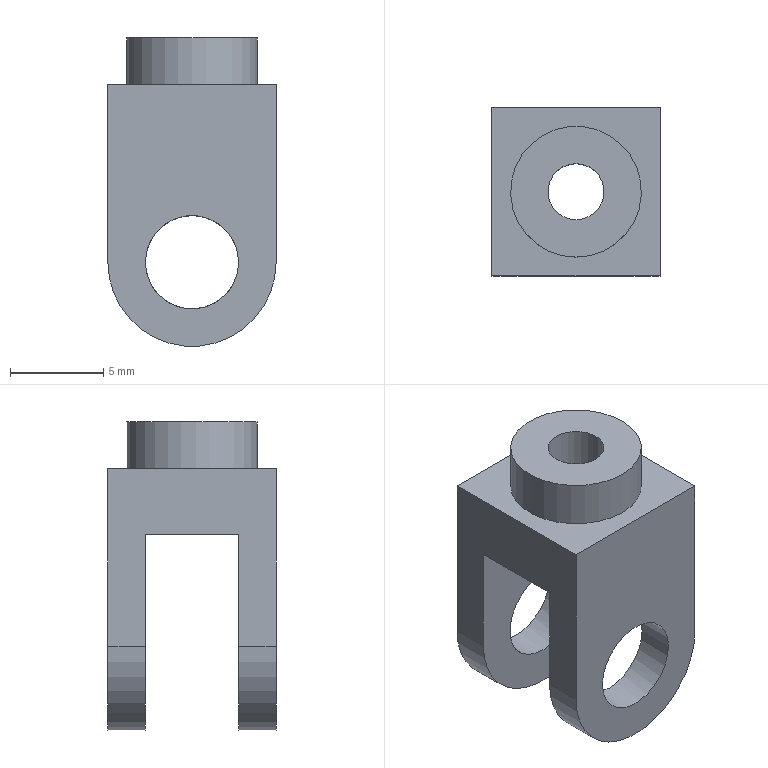Component | NX | CONN_BLOCK | 1 solid | 15 faces | box 9 x 9 x 16.5 mm | volume 602 mm3 | plane 9 | cylinder 6 | commonest cylinder face diameters 9 x2 5 x2 7 x1 3 x1
STEP:
#1=CARTESIAN_POINT('',(0.,0.,0.));
#2=DIRECTION('',(0.,0.,1.));
#3=DIRECTION('',(1.,0.,0.));
#4=AXIS2_PLACEMENT_3D('',#1,#2,#3);
#5=CARTESIAN_POINT('',(-4.5,18.5,86.631));
#6=VERTEX_POINT('',#5);
#7=CARTESIAN_POINT('',(-4.5,20.5,86.631));
#8=VERTEX_POINT('',#7);
#9=CARTESIAN_POINT('',(-4.5,18.5,86.631));
#10=DIRECTION('',(0.,1.,0.));
#11=VECTOR('',#10,1.);
#12=LINE('',#9,#11);
#13=CARTESIAN_POINT('',(-0.,18.5,86.631));
#14=DIRECTION('',(0.,1.,0.));
#15=DIRECTION('',(0.,0.,1.));
#16=AXIS2_PLACEMENT_3D('',#13,#14,#15);
#17=CYLINDRICAL_SURFACE('',#16,4.5);
#18=CARTESIAN_POINT('',(4.712,0.));
#19=DIRECTION('',(0.,1.));
#20=VECTOR('',#19,1.);
#21=LINE('',#18,#20);
#22=(GEOMETRIC_REPRESENTATION_CONTEXT(2)PARAMETRIC_REPRESENTATION_CONTEXT()REPRESENTATION_CONTEXT('',''));
#23=DEFINITIONAL_REPRESENTATION('',(#21),#22);
#24=PCURVE('',#17,#23);
#25=CARTESIAN_POINT('',(-4.5,18.5,96.131));
#26=DIRECTION('',(1.,0.,0.));
#27=DIRECTION('',(-0.,0.,1.));
#28=AXIS2_PLACEMENT_3D('',#25,#26,#27);
#29=PLANE('',#28);
#30=CARTESIAN_POINT('',(-9.5,0.));
#31=DIRECTION('',(0.,-1.));
#32=VECTOR('',#31,1.);
#33=LINE('',#30,#32);
#34=(GEOMETRIC_REPRESENTATION_CONTEXT(2)PARAMETRIC_REPRESENTATION_CONTEXT()REPRESENTATION_CONTEXT('',''));
#35=DEFINITIONAL_REPRESENTATION('',(#33),#34);
#36=PCURVE('',#29,#35);
#37=SURFACE_CURVE('',#12,(#24,#36),.PCURVE_S1.);
#38=EDGE_CURVE('',#6,#8,#37,.T.);
#39=ORIENTED_EDGE('',*,*,#38,.T.);
#40=CARTESIAN_POINT('',(4.5,20.5,86.631));
#41=VERTEX_POINT('',#40);
#42=CARTESIAN_POINT('',(-0.,20.5,86.631));
#43=DIRECTION('',(0.,-1.,-0.));
#44=DIRECTION('',(0.,0.,-1.));
#45=AXIS2_PLACEMENT_3D('',#42,#43,#44);
#46=CIRCLE('',#45,4.5);
#47=CARTESIAN_POINT('',(9.425,2.));
#48=DIRECTION('',(-1.,0.));
#49=VECTOR('',#48,1.);
#50=LINE('',#47,#49);
#51=(GEOMETRIC_REPRESENTATION_CONTEXT(2)PARAMETRIC_REPRESENTATION_CONTEXT()REPRESENTATION_CONTEXT('',''));
#52=DEFINITIONAL_REPRESENTATION('',(#50),#51);
#53=PCURVE('',#17,#52);
#54=CARTESIAN_POINT('',(-5.,20.5,92.631));
#55=DIRECTION('',(0.,-1.,-0.));
#56=DIRECTION('',(0.,0.,-1.));
#57=AXIS2_PLACEMENT_3D('',#54,#55,#56);
#58=PLANE('',#57);
#59=CARTESIAN_POINT('',(6.,5.));
#60=DIRECTION('',(1.,0.));
#61=AXIS2_PLACEMENT_2D('',#59,#60);
#62=CIRCLE('',#61,4.5);
#63=(GEOMETRIC_REPRESENTATION_CONTEXT(2)PARAMETRIC_REPRESENTATION_CONTEXT()REPRESENTATION_CONTEXT('',''));
#64=DEFINITIONAL_REPRESENTATION('',(#62),#63);
#65=PCURVE('',#58,#64);
#66=SURFACE_CURVE('',#46,(#53,#65),.PCURVE_S1.);
#67=EDGE_CURVE('',#8,#41,#66,.T.);
#68=ORIENTED_EDGE('',*,*,#67,.T.);
#69=CARTESIAN_POINT('',(4.5,18.5,86.631));
#70=VERTEX_POINT('',#69);
#71=CARTESIAN_POINT('',(4.5,18.5,86.631));
#72=DIRECTION('',(0.,1.,0.));
#73=VECTOR('',#72,1.);
#74=LINE('',#71,#73);
#75=CARTESIAN_POINT('',(1.571,0.));
#76=DIRECTION('',(0.,1.));
#77=VECTOR('',#76,1.);
#78=LINE('',#75,#77);
#79=(GEOMETRIC_REPRESENTATION_CONTEXT(2)PARAMETRIC_REPRESENTATION_CONTEXT()REPRESENTATION_CONTEXT('',''));
#80=DEFINITIONAL_REPRESENTATION('',(#78),#79);
#81=PCURVE('',#17,#80);
#82=CARTESIAN_POINT('',(4.5,18.5,86.631));
#83=DIRECTION('',(-1.,0.,0.));
#84=DIRECTION('',(-0.,0.,-1.));
#85=AXIS2_PLACEMENT_3D('',#82,#83,#84);
#86=PLANE('',#85);
#87=CARTESIAN_POINT('',(0.,0.));
#88=DIRECTION('',(0.,-1.));
#89=VECTOR('',#88,1.);
#90=LINE('',#87,#89);
#91=(GEOMETRIC_REPRESENTATION_CONTEXT(2)PARAMETRIC_REPRESENTATION_CONTEXT()REPRESENTATION_CONTEXT('',''));
#92=DEFINITIONAL_REPRESENTATION('',(#90),#91);
#93=PCURVE('',#86,#92);
#94=SURFACE_CURVE('',#74,(#81,#93),.PCURVE_S1.);
#95=EDGE_CURVE('',#70,#41,#94,.T.);
#96=ORIENTED_EDGE('',*,*,#95,.F.);
#97=CARTESIAN_POINT('',(-0.,18.5,86.631));
#98=DIRECTION('',(0.,-1.,0.));
#99=DIRECTION('',(1.,0.,0.));
#100=AXIS2_PLACEMENT_3D('',#97,#98,#99);
#101=CIRCLE('',#100,4.5);
#102=CARTESIAN_POINT('',(7.854,0.));
#103=DIRECTION('',(-1.,0.));
#104=VECTOR('',#103,1.);
#105=LINE('',#102,#104);
#106=(GEOMETRIC_REPRESENTATION_CONTEXT(2)PARAMETRIC_REPRESENTATION_CONTEXT()REPRESENTATION_CONTEXT('',''));
#107=DEFINITIONAL_REPRESENTATION('',(#105),#106);
#108=PCURVE('',#17,#107);
#109=CARTESIAN_POINT('',(-0.,18.5,86.631));
#110=DIRECTION('',(0.,-1.,0.));
#111=DIRECTION('',(0.,0.,-1.));
#112=AXIS2_PLACEMENT_3D('',#109,#110,#111);
#113=PLANE('',#112);
#114=CARTESIAN_POINT('',(0.,0.));
#115=DIRECTION('',(0.,1.));
#116=AXIS2_PLACEMENT_2D('',#114,#115);
#117=CIRCLE('',#116,4.5);
#118=(GEOMETRIC_REPRESENTATION_CONTEXT(2)PARAMETRIC_REPRESENTATION_CONTEXT()REPRESENTATION_CONTEXT('',''));
#119=DEFINITIONAL_REPRESENTATION('',(#117),#118);
#120=PCURVE('',#113,#119);
#121=SURFACE_CURVE('',#101,(#108,#120),.PCURVE_S1.);
#122=EDGE_CURVE('',#6,#70,#121,.T.);
#123=ORIENTED_EDGE('',*,*,#122,.F.);
#124=EDGE_LOOP('',(#39,#68,#96,#123));
#125=FACE_BOUND('',#124,.T.);
#126=ADVANCED_FACE('',(#125),#17,.T.);
#127=CARTESIAN_POINT('',(-0.,25.5,89.131));
#128=VERTEX_POINT('',#127);
#129=CARTESIAN_POINT('',(-0.,25.5,86.631));
#130=DIRECTION('',(0.,1.,-0.));
#131=DIRECTION('',(0.,0.,1.));
#132=AXIS2_PLACEMENT_3D('',#129,#130,#131);
#133=CIRCLE('',#132,2.5);
#134=CARTESIAN_POINT('',(-0.,18.5,86.631));
#135=DIRECTION('',(0.,1.,0.));
#136=DIRECTION('',(0.,0.,1.));
#137=AXIS2_PLACEMENT_3D('',#134,#135,#136);
#138=CYLINDRICAL_SURFACE('',#137,2.5);
#139=CARTESIAN_POINT('',(0.,7.));
#140=DIRECTION('',(1.,0.));
#141=VECTOR('',#140,1.);
#142=LINE('',#139,#141);
#143=(GEOMETRIC_REPRESENTATION_CONTEXT(2)PARAMETRIC_REPRESENTATION_CONTEXT()REPRESENTATION_CONTEXT('',''));
#144=DEFINITIONAL_REPRESENTATION('',(#142),#143);
#145=PCURVE('',#138,#144);
#146=CARTESIAN_POINT('',(-5.,25.5,82.131));
#147=DIRECTION('',(0.,1.,-0.));
#148=DIRECTION('',(0.,0.,1.));
#149=AXIS2_PLACEMENT_3D('',#146,#147,#148);
#150=PLANE('',#149);
#151=CARTESIAN_POINT('',(4.5,5.));
#152=DIRECTION('',(1.,0.));
#153=AXIS2_PLACEMENT_2D('',#151,#152);
#154=CIRCLE('',#153,2.5);
#155=(GEOMETRIC_REPRESENTATION_CONTEXT(2)PARAMETRIC_REPRESENTATION_CONTEXT()REPRESENTATION_CONTEXT('',''));
#156=DEFINITIONAL_REPRESENTATION('',(#154),#155);
#157=PCURVE('',#150,#156);
#158=SURFACE_CURVE('',#133,(#145,#157),.PCURVE_S1.);
#159=EDGE_CURVE('',#128,#128,#158,.T.);
#160=ORIENTED_EDGE('',*,*,#159,.T.);
#161=CARTESIAN_POINT('',(-0.,27.5,89.131));
#162=VERTEX_POINT('',#161);
#163=CARTESIAN_POINT('',(-0.,25.5,89.131));
#164=CARTESIAN_POINT('',(-0.,27.5,89.131));
#165=B_SPLINE_CURVE_WITH_KNOTS('',1,(#163,#164),.UNSPECIFIED.,.F.,.F.,(2,2),(7.,9.),.PIECEWISE_BEZIER_KNOTS.);
#166=CARTESIAN_POINT('',(6.283,0.));
#167=DIRECTION('',(0.,1.));
#168=VECTOR('',#167,1.);
#169=LINE('',#166,#168);
#170=(GEOMETRIC_REPRESENTATION_CONTEXT(2)PARAMETRIC_REPRESENTATION_CONTEXT()REPRESENTATION_CONTEXT('',''));
#171=DEFINITIONAL_REPRESENTATION('',(#169),#170);
#172=PCURVE('',#138,#171);
#173=CARTESIAN_POINT('',(0.,0.));
#174=DIRECTION('',(0.,1.));
#175=VECTOR('',#174,1.);
#176=LINE('',#173,#175);
#177=(GEOMETRIC_REPRESENTATION_CONTEXT(2)PARAMETRIC_REPRESENTATION_CONTEXT()REPRESENTATION_CONTEXT('',''));
#178=DEFINITIONAL_REPRESENTATION('',(#176),#177);
#179=PCURVE('',#138,#178);
#180=SEAM_CURVE('',#165,(#172,#179),.PCURVE_S1.);
#181=EDGE_CURVE('',#128,#162,#180,.T.);
#182=ORIENTED_EDGE('',*,*,#181,.T.);
#183=CARTESIAN_POINT('',(2.5,27.5,86.631));
#184=VERTEX_POINT('',#183);
#185=CARTESIAN_POINT('',(-0.,27.5,86.631));
#186=DIRECTION('',(0.,-1.,0.));
#187=DIRECTION('',(1.,0.,0.));
#188=AXIS2_PLACEMENT_3D('',#185,#186,#187);
#189=CIRCLE('',#188,2.5);
#190=CARTESIAN_POINT('',(7.854,9.));
#191=DIRECTION('',(-1.,0.));
#192=VECTOR('',#191,1.);
#193=LINE('',#190,#192);
#194=(GEOMETRIC_REPRESENTATION_CONTEXT(2)PARAMETRIC_REPRESENTATION_CONTEXT()REPRESENTATION_CONTEXT('',''));
#195=DEFINITIONAL_REPRESENTATION('',(#193),#194);
#196=PCURVE('',#138,#195);
#197=CARTESIAN_POINT('',(-0.,27.5,86.631));
#198=DIRECTION('',(0.,-1.,0.));
#199=DIRECTION('',(0.,0.,-1.));
#200=AXIS2_PLACEMENT_3D('',#197,#198,#199);
#201=PLANE('',#200);
#202=CARTESIAN_POINT('',(0.,0.));
#203=DIRECTION('',(0.,1.));
#204=AXIS2_PLACEMENT_2D('',#202,#203);
#205=CIRCLE('',#204,2.5);
#206=(GEOMETRIC_REPRESENTATION_CONTEXT(2)PARAMETRIC_REPRESENTATION_CONTEXT()REPRESENTATION_CONTEXT('',''));
#207=DEFINITIONAL_REPRESENTATION('',(#205),#206);
#208=PCURVE('',#201,#207);
#209=SURFACE_CURVE('',#189,(#196,#208),.PCURVE_S1.);
#210=EDGE_CURVE('',#162,#184,#209,.T.);
#211=ORIENTED_EDGE('',*,*,#210,.T.);
#212=CARTESIAN_POINT('',(-0.,27.5,86.631));
#213=DIRECTION('',(0.,-1.,0.));
#214=DIRECTION('',(1.,0.,0.));
#215=AXIS2_PLACEMENT_3D('',#212,#213,#214);
#216=CIRCLE('',#215,2.5);
#217=CARTESIAN_POINT('',(1.571,9.));
#218=DIRECTION('',(-1.,0.));
#219=VECTOR('',#218,1.);
#220=LINE('',#217,#219);
#221=(GEOMETRIC_REPRESENTATION_CONTEXT(2)PARAMETRIC_REPRESENTATION_CONTEXT()REPRESENTATION_CONTEXT('',''));
#222=DEFINITIONAL_REPRESENTATION('',(#220),#221);
#223=PCURVE('',#138,#222);
#224=CARTESIAN_POINT('',(0.,0.));
#225=DIRECTION('',(0.,1.));
#226=AXIS2_PLACEMENT_2D('',#224,#225);
#227=CIRCLE('',#226,2.5);
#228=(GEOMETRIC_REPRESENTATION_CONTEXT(2)PARAMETRIC_REPRESENTATION_CONTEXT()REPRESENTATION_CONTEXT('',''));
#229=DEFINITIONAL_REPRESENTATION('',(#227),#228);
#230=PCURVE('',#201,#229);
#231=SURFACE_CURVE('',#216,(#223,#230),.PCURVE_S1.);
#232=EDGE_CURVE('',#184,#162,#231,.T.);
#233=ORIENTED_EDGE('',*,*,#232,.T.);
#234=ORIENTED_EDGE('',*,*,#181,.F.);
#235=EDGE_LOOP('',(#160,#182,#211,#233,#234));
#236=FACE_BOUND('',#235,.F.);
#237=ADVANCED_FACE('',(#236),#138,.F.);
#238=CARTESIAN_POINT('',(-0.,21.5,98.631));
#239=VERTEX_POINT('',#238);
#240=CARTESIAN_POINT('',(-0.,23.,98.631));
#241=DIRECTION('',(0.,0.,-1.));
#242=DIRECTION('',(0.,-1.,0.));
#243=AXIS2_PLACEMENT_3D('',#240,#241,#242);
#244=CIRCLE('',#243,1.5);
#245=CARTESIAN_POINT('',(-0.,23.,98.631));
#246=DIRECTION('',(0.,0.,1.));
#247=DIRECTION('',(0.,-1.,0.));
#248=AXIS2_PLACEMENT_3D('',#245,#246,#247);
#249=PLANE('',#248);
#250=CARTESIAN_POINT('',(1.5,0.));
#251=CARTESIAN_POINT('',(1.5,-2.598));
#252=CARTESIAN_POINT('',(-0.75,-1.299));
#253=CARTESIAN_POINT('',(-3.,-0.));
#254=CARTESIAN_POINT('',(-0.75,1.299));
#255=CARTESIAN_POINT('',(1.5,2.598));
#256=CARTESIAN_POINT('',(1.5,0.));
#257=(BOUNDED_CURVE()B_SPLINE_CURVE(2,(#250,#251,#252,#253,#254,#255,#256),.UNSPECIFIED.,.T.,.F.)B_SPLINE_CURVE_WITH_KNOTS((1,2,2,2,2,1),(-2.094,0.,2.094,4.189,6.283,8.378),.UNSPECIFIED.)CURVE()GEOMETRIC_REPRESENTATION_ITEM()RATIONAL_B_SPLINE_CURVE((1.,0.5,1.,0.5,1.,0.5,1.))REPRESENTATION_ITEM(''));
#258=(GEOMETRIC_REPRESENTATION_CONTEXT(2)PARAMETRIC_REPRESENTATION_CONTEXT()REPRESENTATION_CONTEXT('',''));
#259=DEFINITIONAL_REPRESENTATION('',(#257),#258);
#260=PCURVE('',#249,#259);
#261=CARTESIAN_POINT('',(-0.,23.,88.131));
#262=DIRECTION('',(0.,0.,1.));
#263=DIRECTION('',(0.,-1.,0.));
#264=AXIS2_PLACEMENT_3D('',#261,#262,#263);
#265=CYLINDRICAL_SURFACE('',#264,1.5);
#266=CARTESIAN_POINT('',(6.283,10.5));
#267=DIRECTION('',(-1.,0.));
#268=VECTOR('',#267,1.);
#269=LINE('',#266,#268);
#270=(GEOMETRIC_REPRESENTATION_CONTEXT(2)PARAMETRIC_REPRESENTATION_CONTEXT()REPRESENTATION_CONTEXT('',''));
#271=DEFINITIONAL_REPRESENTATION('',(#269),#270);
#272=PCURVE('',#265,#271);
#273=SURFACE_CURVE('',#244,(#260,#272),.PCURVE_S1.);
#274=EDGE_CURVE('',#239,#239,#273,.T.);
#275=ORIENTED_EDGE('',*,*,#274,.T.);
#276=EDGE_LOOP('',(#275));
#277=FACE_BOUND('',#276,.T.);
#278=CARTESIAN_POINT('',(-0.,19.5,98.631));
#279=VERTEX_POINT('',#278);
#280=CARTESIAN_POINT('',(-0.,23.,98.631));
#281=DIRECTION('',(0.,0.,-1.));
#282=DIRECTION('',(0.,-1.,0.));
#283=AXIS2_PLACEMENT_3D('',#280,#281,#282);
#284=CIRCLE('',#283,3.5);
#285=CARTESIAN_POINT('',(3.5,0.));
#286=CARTESIAN_POINT('',(3.5,-6.062));
#287=CARTESIAN_POINT('',(-1.75,-3.031));
#288=CARTESIAN_POINT('',(-7.,-0.));
#289=CARTESIAN_POINT('',(-1.75,3.031));
#290=CARTESIAN_POINT('',(3.5,6.062));
#291=CARTESIAN_POINT('',(3.5,0.));
#292=(BOUNDED_CURVE()B_SPLINE_CURVE(2,(#285,#286,#287,#288,#289,#290,#291),.UNSPECIFIED.,.T.,.F.)B_SPLINE_CURVE_WITH_KNOTS((1,2,2,2,2,1),(-2.094,0.,2.094,4.189,6.283,8.378),.UNSPECIFIED.)CURVE()GEOMETRIC_REPRESENTATION_ITEM()RATIONAL_B_SPLINE_CURVE((1.,0.5,1.,0.5,1.,0.5,1.))REPRESENTATION_ITEM(''));
#293=(GEOMETRIC_REPRESENTATION_CONTEXT(2)PARAMETRIC_REPRESENTATION_CONTEXT()REPRESENTATION_CONTEXT('',''));
#294=DEFINITIONAL_REPRESENTATION('',(#292),#293);
#295=PCURVE('',#249,#294);
#296=CARTESIAN_POINT('',(-0.,23.,96.131));
#297=DIRECTION('',(0.,0.,1.));
#298=DIRECTION('',(0.,-1.,0.));
#299=AXIS2_PLACEMENT_3D('',#296,#297,#298);
#300=CYLINDRICAL_SURFACE('',#299,3.5);
#301=CARTESIAN_POINT('',(6.283,2.5));
#302=DIRECTION('',(-1.,0.));
#303=VECTOR('',#302,1.);
#304=LINE('',#301,#303);
#305=(GEOMETRIC_REPRESENTATION_CONTEXT(2)PARAMETRIC_REPRESENTATION_CONTEXT()REPRESENTATION_CONTEXT('',''));
#306=DEFINITIONAL_REPRESENTATION('',(#304),#305);
#307=PCURVE('',#300,#306);
#308=SURFACE_CURVE('',#284,(#295,#307),.PCURVE_S1.);
#309=EDGE_CURVE('',#279,#279,#308,.T.);
#310=ORIENTED_EDGE('',*,*,#309,.F.);
#311=EDGE_LOOP('',(#310));
#312=FACE_BOUND('',#311,.T.);
#313=ADVANCED_FACE('',(#277,#312),#249,.T.);
#314=ORIENTED_EDGE('',*,*,#309,.T.);
#315=CARTESIAN_POINT('',(-0.,19.5,96.131));
#316=VERTEX_POINT('',#315);
#317=CARTESIAN_POINT('',(-0.,19.5,96.131));
#318=CARTESIAN_POINT('',(-0.,19.5,98.631));
#319=B_SPLINE_CURVE_WITH_KNOTS('',1,(#317,#318),.UNSPECIFIED.,.F.,.F.,(2,2),(0.,2.5),.PIECEWISE_BEZIER_KNOTS.);
#320=CARTESIAN_POINT('',(0.,0.));
#321=DIRECTION('',(0.,1.));
#322=VECTOR('',#321,1.);
#323=LINE('',#320,#322);
#324=(GEOMETRIC_REPRESENTATION_CONTEXT(2)PARAMETRIC_REPRESENTATION_CONTEXT()REPRESENTATION_CONTEXT('',''));
#325=DEFINITIONAL_REPRESENTATION('',(#323),#324);
#326=PCURVE('',#300,#325);
#327=CARTESIAN_POINT('',(6.283,0.));
#328=DIRECTION('',(0.,1.));
#329=VECTOR('',#328,1.);
#330=LINE('',#327,#329);
#331=(GEOMETRIC_REPRESENTATION_CONTEXT(2)PARAMETRIC_REPRESENTATION_CONTEXT()REPRESENTATION_CONTEXT('',''));
#332=DEFINITIONAL_REPRESENTATION('',(#330),#331);
#333=PCURVE('',#300,#332);
#334=SEAM_CURVE('',#319,(#326,#333),.PCURVE_S1.);
#335=EDGE_CURVE('',#316,#279,#334,.T.);
#336=ORIENTED_EDGE('',*,*,#335,.F.);
#337=CARTESIAN_POINT('',(-0.,23.,96.131));
#338=DIRECTION('',(0.,0.,1.));
#339=DIRECTION('',(0.,-1.,0.));
#340=AXIS2_PLACEMENT_3D('',#337,#338,#339);
#341=CIRCLE('',#340,3.5);
#342=CARTESIAN_POINT('',(0.,0.));
#343=DIRECTION('',(1.,0.));
#344=VECTOR('',#343,1.);
#345=LINE('',#342,#344);
#346=(GEOMETRIC_REPRESENTATION_CONTEXT(2)PARAMETRIC_REPRESENTATION_CONTEXT()REPRESENTATION_CONTEXT('',''));
#347=DEFINITIONAL_REPRESENTATION('',(#345),#346);
#348=PCURVE('',#300,#347);
#349=CARTESIAN_POINT('',(-0.,18.5,96.131));
#350=DIRECTION('',(0.,0.,-1.));
#351=DIRECTION('',(0.,1.,0.));
#352=AXIS2_PLACEMENT_3D('',#349,#350,#351);
#353=PLANE('',#352);
#354=CARTESIAN_POINT('',(1.,0.));
#355=CARTESIAN_POINT('',(1.,6.062));
#356=CARTESIAN_POINT('',(6.25,3.031));
#357=CARTESIAN_POINT('',(11.5,0.));
#358=CARTESIAN_POINT('',(6.25,-3.031));
#359=CARTESIAN_POINT('',(1.,-6.062));
#360=CARTESIAN_POINT('',(1.,0.));
#361=(BOUNDED_CURVE()B_SPLINE_CURVE(2,(#354,#355,#356,#357,#358,#359,#360),.UNSPECIFIED.,.T.,.F.)B_SPLINE_CURVE_WITH_KNOTS((1,2,2,2,2,1),(-2.094,0.,2.094,4.189,6.283,8.378),.UNSPECIFIED.)CURVE()GEOMETRIC_REPRESENTATION_ITEM()RATIONAL_B_SPLINE_CURVE((1.,0.5,1.,0.5,1.,0.5,1.))REPRESENTATION_ITEM(''));
#362=(GEOMETRIC_REPRESENTATION_CONTEXT(2)PARAMETRIC_REPRESENTATION_CONTEXT()REPRESENTATION_CONTEXT('',''));
#363=DEFINITIONAL_REPRESENTATION('',(#361),#362);
#364=PCURVE('',#353,#363);
#365=SURFACE_CURVE('',#341,(#348,#364),.PCURVE_S1.);
#366=EDGE_CURVE('',#316,#316,#365,.T.);
#367=ORIENTED_EDGE('',*,*,#366,.T.);
#368=ORIENTED_EDGE('',*,*,#335,.T.);
#369=EDGE_LOOP('',(#314,#336,#367,#368));
#370=FACE_BOUND('',#369,.T.);
#371=ADVANCED_FACE('',(#370),#300,.T.);
#372=CARTESIAN_POINT('',(4.5,25.5,86.631));
#373=VERTEX_POINT('',#372);
#374=CARTESIAN_POINT('',(-4.5,25.5,86.631));
#375=VERTEX_POINT('',#374);
#376=CARTESIAN_POINT('',(-0.,25.5,86.631));
#377=DIRECTION('',(0.,1.,-0.));
#378=DIRECTION('',(0.,0.,1.));
#379=AXIS2_PLACEMENT_3D('',#376,#377,#378);
#380=CIRCLE('',#379,4.5);
#381=CARTESIAN_POINT('',(-0.,18.5,86.631));
#382=DIRECTION('',(0.,1.,0.));
#383=DIRECTION('',(0.,0.,1.));
#384=AXIS2_PLACEMENT_3D('',#381,#382,#383);
#385=CYLINDRICAL_SURFACE('',#384,4.5);
#386=CARTESIAN_POINT('',(0.,7.));
#387=DIRECTION('',(1.,0.));
#388=VECTOR('',#387,1.);
#389=LINE('',#386,#388);
#390=(GEOMETRIC_REPRESENTATION_CONTEXT(2)PARAMETRIC_REPRESENTATION_CONTEXT()REPRESENTATION_CONTEXT('',''));
#391=DEFINITIONAL_REPRESENTATION('',(#389),#390);
#392=PCURVE('',#385,#391);
#393=CARTESIAN_POINT('',(4.5,5.));
#394=DIRECTION('',(1.,0.));
#395=AXIS2_PLACEMENT_2D('',#393,#394);
#396=CIRCLE('',#395,4.5);
#397=(GEOMETRIC_REPRESENTATION_CONTEXT(2)PARAMETRIC_REPRESENTATION_CONTEXT()REPRESENTATION_CONTEXT('',''));
#398=DEFINITIONAL_REPRESENTATION('',(#396),#397);
#399=PCURVE('',#150,#398);
#400=SURFACE_CURVE('',#380,(#392,#399),.PCURVE_S1.);
#401=EDGE_CURVE('',#373,#375,#400,.T.);
#402=ORIENTED_EDGE('',*,*,#401,.T.);
#403=CARTESIAN_POINT('',(-4.5,27.5,86.631));
#404=VERTEX_POINT('',#403);
#405=CARTESIAN_POINT('',(-4.5,18.5,86.631));
#406=DIRECTION('',(0.,1.,0.));
#407=VECTOR('',#406,1.);
#408=LINE('',#405,#407);
#409=CARTESIAN_POINT('',(4.712,0.));
#410=DIRECTION('',(0.,1.));
#411=VECTOR('',#410,1.);
#412=LINE('',#409,#411);
#413=(GEOMETRIC_REPRESENTATION_CONTEXT(2)PARAMETRIC_REPRESENTATION_CONTEXT()REPRESENTATION_CONTEXT('',''));
#414=DEFINITIONAL_REPRESENTATION('',(#412),#413);
#415=PCURVE('',#385,#414);
#416=CARTESIAN_POINT('',(-9.5,0.));
#417=DIRECTION('',(0.,-1.));
#418=VECTOR('',#417,1.);
#419=LINE('',#416,#418);
#420=(GEOMETRIC_REPRESENTATION_CONTEXT(2)PARAMETRIC_REPRESENTATION_CONTEXT()REPRESENTATION_CONTEXT('',''));
#421=DEFINITIONAL_REPRESENTATION('',(#419),#420);
#422=PCURVE('',#29,#421);
#423=SURFACE_CURVE('',#408,(#415,#422),.PCURVE_S1.);
#424=EDGE_CURVE('',#375,#404,#423,.T.);
#425=ORIENTED_EDGE('',*,*,#424,.T.);
#426=CARTESIAN_POINT('',(4.5,27.5,86.631));
#427=VERTEX_POINT('',#426);
#428=CARTESIAN_POINT('',(-0.,27.5,86.631));
#429=DIRECTION('',(0.,-1.,0.));
#430=DIRECTION('',(1.,0.,0.));
#431=AXIS2_PLACEMENT_3D('',#428,#429,#430);
#432=CIRCLE('',#431,4.5);
#433=CARTESIAN_POINT('',(7.854,9.));
#434=DIRECTION('',(-1.,0.));
#435=VECTOR('',#434,1.);
#436=LINE('',#433,#435);
#437=(GEOMETRIC_REPRESENTATION_CONTEXT(2)PARAMETRIC_REPRESENTATION_CONTEXT()REPRESENTATION_CONTEXT('',''));
#438=DEFINITIONAL_REPRESENTATION('',(#436),#437);
#439=PCURVE('',#385,#438);
#440=CARTESIAN_POINT('',(0.,0.));
#441=DIRECTION('',(0.,1.));
#442=AXIS2_PLACEMENT_2D('',#440,#441);
#443=CIRCLE('',#442,4.5);
#444=(GEOMETRIC_REPRESENTATION_CONTEXT(2)PARAMETRIC_REPRESENTATION_CONTEXT()REPRESENTATION_CONTEXT('',''));
#445=DEFINITIONAL_REPRESENTATION('',(#443),#444);
#446=PCURVE('',#201,#445);
#447=SURFACE_CURVE('',#432,(#439,#446),.PCURVE_S1.);
#448=EDGE_CURVE('',#404,#427,#447,.T.);
#449=ORIENTED_EDGE('',*,*,#448,.T.);
#450=CARTESIAN_POINT('',(4.5,18.5,86.631));
#451=DIRECTION('',(0.,1.,0.));
#452=VECTOR('',#451,1.);
#453=LINE('',#450,#452);
#454=CARTESIAN_POINT('',(1.571,0.));
#455=DIRECTION('',(0.,1.));
#456=VECTOR('',#455,1.);
#457=LINE('',#454,#456);
#458=(GEOMETRIC_REPRESENTATION_CONTEXT(2)PARAMETRIC_REPRESENTATION_CONTEXT()REPRESENTATION_CONTEXT('',''));
#459=DEFINITIONAL_REPRESENTATION('',(#457),#458);
#460=PCURVE('',#385,#459);
#461=CARTESIAN_POINT('',(0.,0.));
#462=DIRECTION('',(0.,-1.));
#463=VECTOR('',#462,1.);
#464=LINE('',#461,#463);
#465=(GEOMETRIC_REPRESENTATION_CONTEXT(2)PARAMETRIC_REPRESENTATION_CONTEXT()REPRESENTATION_CONTEXT('',''));
#466=DEFINITIONAL_REPRESENTATION('',(#464),#465);
#467=PCURVE('',#86,#466);
#468=SURFACE_CURVE('',#453,(#460,#467),.PCURVE_S1.);
#469=EDGE_CURVE('',#373,#427,#468,.T.);
#470=ORIENTED_EDGE('',*,*,#469,.F.);
#471=EDGE_LOOP('',(#402,#425,#449,#470));
#472=FACE_BOUND('',#471,.T.);
#473=ADVANCED_FACE('',(#472),#385,.T.);
#474=CARTESIAN_POINT('',(4.5,20.5,92.631));
#475=VERTEX_POINT('',#474);
#476=CARTESIAN_POINT('',(4.5,25.5,92.631));
#477=VERTEX_POINT('',#476);
#478=CARTESIAN_POINT('',(4.5,18.5,92.631));
#479=DIRECTION('',(0.,1.,0.));
#480=VECTOR('',#479,1.);
#481=LINE('',#478,#480);
#482=CARTESIAN_POINT('',(-6.,0.));
#483=DIRECTION('',(0.,-1.));
#484=VECTOR('',#483,1.);
#485=LINE('',#482,#484);
#486=(GEOMETRIC_REPRESENTATION_CONTEXT(2)PARAMETRIC_REPRESENTATION_CONTEXT()REPRESENTATION_CONTEXT('',''));
#487=DEFINITIONAL_REPRESENTATION('',(#485),#486);
#488=PCURVE('',#86,#487);
#489=CARTESIAN_POINT('',(-5.,25.5,92.631));
#490=DIRECTION('',(0.,0.,1.));
#491=DIRECTION('',(0.,-1.,0.));
#492=AXIS2_PLACEMENT_3D('',#489,#490,#491);
#493=PLANE('',#492);
#494=CARTESIAN_POINT('',(7.,9.5));
#495=DIRECTION('',(-1.,0.));
#496=VECTOR('',#495,1.);
#497=LINE('',#494,#496);
#498=(GEOMETRIC_REPRESENTATION_CONTEXT(2)PARAMETRIC_REPRESENTATION_CONTEXT()REPRESENTATION_CONTEXT('',''));
#499=DEFINITIONAL_REPRESENTATION('',(#497),#498);
#500=PCURVE('',#493,#499);
#501=SURFACE_CURVE('',#481,(#488,#500),.PCURVE_S1.);
#502=EDGE_CURVE('',#475,#477,#501,.T.);
#503=ORIENTED_EDGE('',*,*,#502,.T.);
#504=CARTESIAN_POINT('',(4.5,25.5,86.631));
#505=DIRECTION('',(-0.,-0.,-1.));
#506=VECTOR('',#505,1.);
#507=LINE('',#504,#506);
#508=CARTESIAN_POINT('',(0.,-7.));
#509=DIRECTION('',(1.,0.));
#510=VECTOR('',#509,1.);
#511=LINE('',#508,#510);
#512=(GEOMETRIC_REPRESENTATION_CONTEXT(2)PARAMETRIC_REPRESENTATION_CONTEXT()REPRESENTATION_CONTEXT('',''));
#513=DEFINITIONAL_REPRESENTATION('',(#511),#512);
#514=PCURVE('',#86,#513);
#515=CARTESIAN_POINT('',(4.5,9.5));
#516=DIRECTION('',(-1.,-0.));
#517=VECTOR('',#516,1.);
#518=LINE('',#515,#517);
#519=(GEOMETRIC_REPRESENTATION_CONTEXT(2)PARAMETRIC_REPRESENTATION_CONTEXT()REPRESENTATION_CONTEXT('',''));
#520=DEFINITIONAL_REPRESENTATION('',(#518),#519);
#521=PCURVE('',#150,#520);
#522=SURFACE_CURVE('',#507,(#514,#521),.PCURVE_S1.);
#523=EDGE_CURVE('',#477,#373,#522,.T.);
#524=ORIENTED_EDGE('',*,*,#523,.T.);
#525=ORIENTED_EDGE('',*,*,#469,.T.);
#526=CARTESIAN_POINT('',(4.5,27.5,96.131));
#527=VERTEX_POINT('',#526);
#528=CARTESIAN_POINT('',(4.5,27.5,86.631));
#529=DIRECTION('',(0.,0.,1.));
#530=VECTOR('',#529,1.);
#531=LINE('',#528,#530);
#532=CARTESIAN_POINT('',(0.,-9.));
#533=DIRECTION('',(-1.,0.));
#534=VECTOR('',#533,1.);
#535=LINE('',#532,#534);
#536=(GEOMETRIC_REPRESENTATION_CONTEXT(2)PARAMETRIC_REPRESENTATION_CONTEXT()REPRESENTATION_CONTEXT('',''));
#537=DEFINITIONAL_REPRESENTATION('',(#535),#536);
#538=PCURVE('',#86,#537);
#539=CARTESIAN_POINT('',(0.,4.5));
#540=DIRECTION('',(-1.,0.));
#541=VECTOR('',#540,1.);
#542=LINE('',#539,#541);
#543=(GEOMETRIC_REPRESENTATION_CONTEXT(2)PARAMETRIC_REPRESENTATION_CONTEXT()REPRESENTATION_CONTEXT('',''));
#544=DEFINITIONAL_REPRESENTATION('',(#542),#543);
#545=PCURVE('',#201,#544);
#546=SURFACE_CURVE('',#531,(#538,#545),.PCURVE_S1.);
#547=EDGE_CURVE('',#427,#527,#546,.T.);
#548=ORIENTED_EDGE('',*,*,#547,.T.);
#549=CARTESIAN_POINT('',(4.5,18.5,96.131));
#550=VERTEX_POINT('',#549);
#551=CARTESIAN_POINT('',(4.5,18.5,96.131));
#552=DIRECTION('',(0.,1.,0.));
#553=VECTOR('',#552,1.);
#554=LINE('',#551,#553);
#555=CARTESIAN_POINT('',(-9.5,0.));
#556=DIRECTION('',(0.,-1.));
#557=VECTOR('',#556,1.);
#558=LINE('',#555,#557);
#559=(GEOMETRIC_REPRESENTATION_CONTEXT(2)PARAMETRIC_REPRESENTATION_CONTEXT()REPRESENTATION_CONTEXT('',''));
#560=DEFINITIONAL_REPRESENTATION('',(#558),#559);
#561=PCURVE('',#86,#560);
#562=CARTESIAN_POINT('',(0.,4.5));
#563=DIRECTION('',(1.,0.));
#564=VECTOR('',#563,1.);
#565=LINE('',#562,#564);
#566=(GEOMETRIC_REPRESENTATION_CONTEXT(2)PARAMETRIC_REPRESENTATION_CONTEXT()REPRESENTATION_CONTEXT('',''));
#567=DEFINITIONAL_REPRESENTATION('',(#565),#566);
#568=PCURVE('',#353,#567);
#569=SURFACE_CURVE('',#554,(#561,#568),.PCURVE_S1.);
#570=EDGE_CURVE('',#550,#527,#569,.T.);
#571=ORIENTED_EDGE('',*,*,#570,.F.);
#572=CARTESIAN_POINT('',(4.5,18.5,86.631));
#573=DIRECTION('',(0.,0.,1.));
#574=VECTOR('',#573,1.);
#575=LINE('',#572,#574);
#576=CARTESIAN_POINT('',(0.,0.));
#577=DIRECTION('',(-1.,0.));
#578=VECTOR('',#577,1.);
#579=LINE('',#576,#578);
#580=(GEOMETRIC_REPRESENTATION_CONTEXT(2)PARAMETRIC_REPRESENTATION_CONTEXT()REPRESENTATION_CONTEXT('',''));
#581=DEFINITIONAL_REPRESENTATION('',(#579),#580);
#582=PCURVE('',#86,#581);
#583=CARTESIAN_POINT('',(0.,4.5));
#584=DIRECTION('',(-1.,0.));
#585=VECTOR('',#584,1.);
#586=LINE('',#583,#585);
#587=(GEOMETRIC_REPRESENTATION_CONTEXT(2)PARAMETRIC_REPRESENTATION_CONTEXT()REPRESENTATION_CONTEXT('',''));
#588=DEFINITIONAL_REPRESENTATION('',(#586),#587);
#589=PCURVE('',#113,#588);
#590=SURFACE_CURVE('',#575,(#582,#589),.PCURVE_S1.);
#591=EDGE_CURVE('',#70,#550,#590,.T.);
#592=ORIENTED_EDGE('',*,*,#591,.F.);
#593=ORIENTED_EDGE('',*,*,#95,.T.);
#594=CARTESIAN_POINT('',(4.5,20.5,86.631));
#595=DIRECTION('',(0.,-0.,1.));
#596=VECTOR('',#595,1.);
#597=LINE('',#594,#596);
#598=CARTESIAN_POINT('',(0.,-2.));
#599=DIRECTION('',(-1.,0.));
#600=VECTOR('',#599,1.);
#601=LINE('',#598,#600);
#602=(GEOMETRIC_REPRESENTATION_CONTEXT(2)PARAMETRIC_REPRESENTATION_CONTEXT()REPRESENTATION_CONTEXT('',''));
#603=DEFINITIONAL_REPRESENTATION('',(#601),#602);
#604=PCURVE('',#86,#603);
#605=CARTESIAN_POINT('',(6.,9.5));
#606=DIRECTION('',(-1.,0.));
#607=VECTOR('',#606,1.);
#608=LINE('',#605,#607);
#609=(GEOMETRIC_REPRESENTATION_CONTEXT(2)PARAMETRIC_REPRESENTATION_CONTEXT()REPRESENTATION_CONTEXT('',''));
#610=DEFINITIONAL_REPRESENTATION('',(#608),#609);
#611=PCURVE('',#58,#610);
#612=SURFACE_CURVE('',#597,(#604,#611),.PCURVE_S1.);
#613=EDGE_CURVE('',#41,#475,#612,.T.);
#614=ORIENTED_EDGE('',*,*,#613,.T.);
#615=EDGE_LOOP('',(#503,#524,#525,#548,#571,#592,#593,#614));
#616=FACE_BOUND('',#615,.T.);
#617=ADVANCED_FACE('',(#616),#86,.F.);
#618=ORIENTED_EDGE('',*,*,#366,.F.);
#619=EDGE_LOOP('',(#618));
#620=FACE_BOUND('',#619,.T.);
#621=CARTESIAN_POINT('',(-4.5,27.5,96.131));
#622=VERTEX_POINT('',#621);
#623=CARTESIAN_POINT('',(-0.,27.5,96.131));
#624=DIRECTION('',(-1.,0.,0.));
#625=VECTOR('',#624,1.);
#626=LINE('',#623,#625);
#627=CARTESIAN_POINT('',(9.,0.));
#628=DIRECTION('',(0.,-1.));
#629=VECTOR('',#628,1.);
#630=LINE('',#627,#629);
#631=(GEOMETRIC_REPRESENTATION_CONTEXT(2)PARAMETRIC_REPRESENTATION_CONTEXT()REPRESENTATION_CONTEXT('',''));
#632=DEFINITIONAL_REPRESENTATION('',(#630),#631);
#633=PCURVE('',#353,#632);
#634=CARTESIAN_POINT('',(-9.5,0.));
#635=DIRECTION('',(0.,-1.));
#636=VECTOR('',#635,1.);
#637=LINE('',#634,#636);
#638=(GEOMETRIC_REPRESENTATION_CONTEXT(2)PARAMETRIC_REPRESENTATION_CONTEXT()REPRESENTATION_CONTEXT('',''));
#639=DEFINITIONAL_REPRESENTATION('',(#637),#638);
#640=PCURVE('',#201,#639);
#641=SURFACE_CURVE('',#626,(#633,#640),.PCURVE_S1.);
#642=EDGE_CURVE('',#527,#622,#641,.T.);
#643=ORIENTED_EDGE('',*,*,#642,.T.);
#644=CARTESIAN_POINT('',(-4.5,18.5,96.131));
#645=VERTEX_POINT('',#644);
#646=CARTESIAN_POINT('',(-4.5,18.5,96.131));
#647=DIRECTION('',(0.,1.,0.));
#648=VECTOR('',#647,1.);
#649=LINE('',#646,#648);
#650=CARTESIAN_POINT('',(0.,-4.5));
#651=DIRECTION('',(1.,0.));
#652=VECTOR('',#651,1.);
#653=LINE('',#650,#652);
#654=(GEOMETRIC_REPRESENTATION_CONTEXT(2)PARAMETRIC_REPRESENTATION_CONTEXT()REPRESENTATION_CONTEXT('',''));
#655=DEFINITIONAL_REPRESENTATION('',(#653),#654);
#656=PCURVE('',#353,#655);
#657=CARTESIAN_POINT('',(0.,0.));
#658=DIRECTION('',(0.,-1.));
#659=VECTOR('',#658,1.);
#660=LINE('',#657,#659);
#661=(GEOMETRIC_REPRESENTATION_CONTEXT(2)PARAMETRIC_REPRESENTATION_CONTEXT()REPRESENTATION_CONTEXT('',''));
#662=DEFINITIONAL_REPRESENTATION('',(#660),#661);
#663=PCURVE('',#29,#662);
#664=SURFACE_CURVE('',#649,(#656,#663),.PCURVE_S1.);
#665=EDGE_CURVE('',#645,#622,#664,.T.);
#666=ORIENTED_EDGE('',*,*,#665,.F.);
#667=CARTESIAN_POINT('',(4.5,18.5,96.131));
#668=DIRECTION('',(-1.,0.,0.));
#669=VECTOR('',#668,1.);
#670=LINE('',#667,#669);
#671=CARTESIAN_POINT('',(0.,4.5));
#672=DIRECTION('',(0.,-1.));
#673=VECTOR('',#672,1.);
#674=LINE('',#671,#673);
#675=(GEOMETRIC_REPRESENTATION_CONTEXT(2)PARAMETRIC_REPRESENTATION_CONTEXT()REPRESENTATION_CONTEXT('',''));
#676=DEFINITIONAL_REPRESENTATION('',(#674),#675);
#677=PCURVE('',#353,#676);
#678=CARTESIAN_POINT('',(-9.5,4.5));
#679=DIRECTION('',(0.,-1.));
#680=VECTOR('',#679,1.);
#681=LINE('',#678,#680);
#682=(GEOMETRIC_REPRESENTATION_CONTEXT(2)PARAMETRIC_REPRESENTATION_CONTEXT()REPRESENTATION_CONTEXT('',''));
#683=DEFINITIONAL_REPRESENTATION('',(#681),#682);
#684=PCURVE('',#113,#683);
#685=SURFACE_CURVE('',#670,(#677,#684),.PCURVE_S1.);
#686=EDGE_CURVE('',#550,#645,#685,.T.);
#687=ORIENTED_EDGE('',*,*,#686,.F.);
#688=ORIENTED_EDGE('',*,*,#570,.T.);
#689=EDGE_LOOP('',(#643,#666,#687,#688));
#690=FACE_BOUND('',#689,.T.);
#691=ADVANCED_FACE('',(#620,#690),#353,.F.);
#692=ORIENTED_EDGE('',*,*,#424,.F.);
#693=CARTESIAN_POINT('',(-4.5,25.5,92.631));
#694=VERTEX_POINT('',#693);
#695=CARTESIAN_POINT('',(-4.5,25.5,96.131));
#696=DIRECTION('',(-0.,0.,1.));
#697=VECTOR('',#696,1.);
#698=LINE('',#695,#697);
#699=CARTESIAN_POINT('',(0.,-7.));
#700=DIRECTION('',(1.,-0.));
#701=VECTOR('',#700,1.);
#702=LINE('',#699,#701);
#703=(GEOMETRIC_REPRESENTATION_CONTEXT(2)PARAMETRIC_REPRESENTATION_CONTEXT()REPRESENTATION_CONTEXT('',''));
#704=DEFINITIONAL_REPRESENTATION('',(#702),#703);
#705=PCURVE('',#29,#704);
#706=CARTESIAN_POINT('',(14.,0.5));
#707=DIRECTION('',(1.,-0.));
#708=VECTOR('',#707,1.);
#709=LINE('',#706,#708);
#710=(GEOMETRIC_REPRESENTATION_CONTEXT(2)PARAMETRIC_REPRESENTATION_CONTEXT()REPRESENTATION_CONTEXT('',''));
#711=DEFINITIONAL_REPRESENTATION('',(#709),#710);
#712=PCURVE('',#150,#711);
#713=SURFACE_CURVE('',#698,(#705,#712),.PCURVE_S1.);
#714=EDGE_CURVE('',#375,#694,#713,.T.);
#715=ORIENTED_EDGE('',*,*,#714,.T.);
#716=CARTESIAN_POINT('',(-4.5,20.5,92.631));
#717=VERTEX_POINT('',#716);
#718=CARTESIAN_POINT('',(-4.5,18.5,92.631));
#719=DIRECTION('',(0.,-1.,0.));
#720=VECTOR('',#719,1.);
#721=LINE('',#718,#720);
#722=CARTESIAN_POINT('',(-3.5,0.));
#723=DIRECTION('',(0.,1.));
#724=VECTOR('',#723,1.);
#725=LINE('',#722,#724);
#726=(GEOMETRIC_REPRESENTATION_CONTEXT(2)PARAMETRIC_REPRESENTATION_CONTEXT()REPRESENTATION_CONTEXT('',''));
#727=DEFINITIONAL_REPRESENTATION('',(#725),#726);
#728=PCURVE('',#29,#727);
#729=CARTESIAN_POINT('',(7.,0.5));
#730=DIRECTION('',(1.,0.));
#731=VECTOR('',#730,1.);
#732=LINE('',#729,#731);
#733=(GEOMETRIC_REPRESENTATION_CONTEXT(2)PARAMETRIC_REPRESENTATION_CONTEXT()REPRESENTATION_CONTEXT('',''));
#734=DEFINITIONAL_REPRESENTATION('',(#732),#733);
#735=PCURVE('',#493,#734);
#736=SURFACE_CURVE('',#721,(#728,#735),.PCURVE_S1.);
#737=EDGE_CURVE('',#694,#717,#736,.T.);
#738=ORIENTED_EDGE('',*,*,#737,.T.);
#739=CARTESIAN_POINT('',(-4.5,20.5,96.131));
#740=DIRECTION('',(0.,0.,-1.));
#741=VECTOR('',#740,1.);
#742=LINE('',#739,#741);
#743=CARTESIAN_POINT('',(0.,-2.));
#744=DIRECTION('',(-1.,-0.));
#745=VECTOR('',#744,1.);
#746=LINE('',#743,#745);
#747=(GEOMETRIC_REPRESENTATION_CONTEXT(2)PARAMETRIC_REPRESENTATION_CONTEXT()REPRESENTATION_CONTEXT('',''));
#748=DEFINITIONAL_REPRESENTATION('',(#746),#747);
#749=PCURVE('',#29,#748);
#750=CARTESIAN_POINT('',(-3.5,0.5));
#751=DIRECTION('',(1.,0.));
#752=VECTOR('',#751,1.);
#753=LINE('',#750,#752);
#754=(GEOMETRIC_REPRESENTATION_CONTEXT(2)PARAMETRIC_REPRESENTATION_CONTEXT()REPRESENTATION_CONTEXT('',''));
#755=DEFINITIONAL_REPRESENTATION('',(#753),#754);
#756=PCURVE('',#58,#755);
#757=SURFACE_CURVE('',#742,(#749,#756),.PCURVE_S1.);
#758=EDGE_CURVE('',#717,#8,#757,.T.);
#759=ORIENTED_EDGE('',*,*,#758,.T.);
#760=ORIENTED_EDGE('',*,*,#38,.F.);
#761=CARTESIAN_POINT('',(-4.5,18.5,96.131));
#762=DIRECTION('',(0.,0.,-1.));
#763=VECTOR('',#762,1.);
#764=LINE('',#761,#763);
#765=CARTESIAN_POINT('',(0.,0.));
#766=DIRECTION('',(-1.,0.));
#767=VECTOR('',#766,1.);
#768=LINE('',#765,#767);
#769=(GEOMETRIC_REPRESENTATION_CONTEXT(2)PARAMETRIC_REPRESENTATION_CONTEXT()REPRESENTATION_CONTEXT('',''));
#770=DEFINITIONAL_REPRESENTATION('',(#768),#769);
#771=PCURVE('',#29,#770);
#772=CARTESIAN_POINT('',(-9.5,-4.5));
#773=DIRECTION('',(1.,0.));
#774=VECTOR('',#773,1.);
#775=LINE('',#772,#774);
#776=(GEOMETRIC_REPRESENTATION_CONTEXT(2)PARAMETRIC_REPRESENTATION_CONTEXT()REPRESENTATION_CONTEXT('',''));
#777=DEFINITIONAL_REPRESENTATION('',(#775),#776);
#778=PCURVE('',#113,#777);
#779=SURFACE_CURVE('',#764,(#771,#778),.PCURVE_S1.);
#780=EDGE_CURVE('',#645,#6,#779,.T.);
#781=ORIENTED_EDGE('',*,*,#780,.F.);
#782=ORIENTED_EDGE('',*,*,#665,.T.);
#783=CARTESIAN_POINT('',(-4.5,27.5,96.131));
#784=DIRECTION('',(0.,0.,-1.));
#785=VECTOR('',#784,1.);
#786=LINE('',#783,#785);
#787=CARTESIAN_POINT('',(0.,-9.));
#788=DIRECTION('',(-1.,0.));
#789=VECTOR('',#788,1.);
#790=LINE('',#787,#789);
#791=(GEOMETRIC_REPRESENTATION_CONTEXT(2)PARAMETRIC_REPRESENTATION_CONTEXT()REPRESENTATION_CONTEXT('',''));
#792=DEFINITIONAL_REPRESENTATION('',(#790),#791);
#793=PCURVE('',#29,#792);
#794=CARTESIAN_POINT('',(-9.5,-4.5));
#795=DIRECTION('',(1.,0.));
#796=VECTOR('',#795,1.);
#797=LINE('',#794,#796);
#798=(GEOMETRIC_REPRESENTATION_CONTEXT(2)PARAMETRIC_REPRESENTATION_CONTEXT()REPRESENTATION_CONTEXT('',''));
#799=DEFINITIONAL_REPRESENTATION('',(#797),#798);
#800=PCURVE('',#201,#799);
#801=SURFACE_CURVE('',#786,(#793,#800),.PCURVE_S1.);
#802=EDGE_CURVE('',#622,#404,#801,.T.);
#803=ORIENTED_EDGE('',*,*,#802,.T.);
#804=EDGE_LOOP('',(#692,#715,#738,#759,#760,#781,#782,#803));
#805=FACE_BOUND('',#804,.T.);
#806=ADVANCED_FACE('',(#805),#29,.F.);
#807=CARTESIAN_POINT('',(-0.,20.5,84.131));
#808=VERTEX_POINT('',#807);
#809=CARTESIAN_POINT('',(2.5,20.5,86.631));
#810=VERTEX_POINT('',#809);
#811=CARTESIAN_POINT('',(-0.,20.5,86.631));
#812=DIRECTION('',(0.,-1.,-0.));
#813=DIRECTION('',(0.,0.,-1.));
#814=AXIS2_PLACEMENT_3D('',#811,#812,#813);
#815=CIRCLE('',#814,2.5);
#816=CARTESIAN_POINT('',(-0.,18.5,86.631));
#817=DIRECTION('',(0.,1.,0.));
#818=DIRECTION('',(0.,0.,1.));
#819=AXIS2_PLACEMENT_3D('',#816,#817,#818);
#820=CYLINDRICAL_SURFACE('',#819,2.5);
#821=CARTESIAN_POINT('',(3.142,2.));
#822=DIRECTION('',(-1.,0.));
#823=VECTOR('',#822,1.);
#824=LINE('',#821,#823);
#825=(GEOMETRIC_REPRESENTATION_CONTEXT(2)PARAMETRIC_REPRESENTATION_CONTEXT()REPRESENTATION_CONTEXT('',''));
#826=DEFINITIONAL_REPRESENTATION('',(#824),#825);
#827=PCURVE('',#820,#826);
#828=CARTESIAN_POINT('',(6.,5.));
#829=DIRECTION('',(1.,0.));
#830=AXIS2_PLACEMENT_2D('',#828,#829);
#831=CIRCLE('',#830,2.5);
#832=(GEOMETRIC_REPRESENTATION_CONTEXT(2)PARAMETRIC_REPRESENTATION_CONTEXT()REPRESENTATION_CONTEXT('',''));
#833=DEFINITIONAL_REPRESENTATION('',(#831),#832);
#834=PCURVE('',#58,#833);
#835=SURFACE_CURVE('',#815,(#827,#834),.PCURVE_S1.);
#836=EDGE_CURVE('',#808,#810,#835,.T.);
#837=ORIENTED_EDGE('',*,*,#836,.T.);
#838=CARTESIAN_POINT('',(2.5,18.5,86.631));
#839=VERTEX_POINT('',#838);
#840=CARTESIAN_POINT('',(2.5,18.5,86.631));
#841=CARTESIAN_POINT('',(2.5,20.5,86.631));
#842=B_SPLINE_CURVE_WITH_KNOTS('',1,(#840,#841),.UNSPECIFIED.,.F.,.F.,(2,2),(0.,2.),.PIECEWISE_BEZIER_KNOTS.);
#843=CARTESIAN_POINT('',(1.571,0.));
#844=DIRECTION('',(0.,1.));
#845=VECTOR('',#844,1.);
#846=LINE('',#843,#845);
#847=(GEOMETRIC_REPRESENTATION_CONTEXT(2)PARAMETRIC_REPRESENTATION_CONTEXT()REPRESENTATION_CONTEXT('',''));
#848=DEFINITIONAL_REPRESENTATION('',(#846),#847);
#849=PCURVE('',#820,#848);
#850=CARTESIAN_POINT('',(7.854,0.));
#851=DIRECTION('',(0.,1.));
#852=VECTOR('',#851,1.);
#853=LINE('',#850,#852);
#854=(GEOMETRIC_REPRESENTATION_CONTEXT(2)PARAMETRIC_REPRESENTATION_CONTEXT()REPRESENTATION_CONTEXT('',''));
#855=DEFINITIONAL_REPRESENTATION('',(#853),#854);
#856=PCURVE('',#820,#855);
#857=SEAM_CURVE('',#842,(#849,#856),.PCURVE_S1.);
#858=EDGE_CURVE('',#839,#810,#857,.T.);
#859=ORIENTED_EDGE('',*,*,#858,.F.);
#860=CARTESIAN_POINT('',(-0.,18.5,86.631));
#861=DIRECTION('',(0.,-1.,0.));
#862=DIRECTION('',(1.,0.,0.));
#863=AXIS2_PLACEMENT_3D('',#860,#861,#862);
#864=CIRCLE('',#863,2.5);
#865=CARTESIAN_POINT('',(7.854,0.));
#866=DIRECTION('',(-1.,0.));
#867=VECTOR('',#866,1.);
#868=LINE('',#865,#867);
#869=(GEOMETRIC_REPRESENTATION_CONTEXT(2)PARAMETRIC_REPRESENTATION_CONTEXT()REPRESENTATION_CONTEXT('',''));
#870=DEFINITIONAL_REPRESENTATION('',(#868),#869);
#871=PCURVE('',#820,#870);
#872=CARTESIAN_POINT('',(0.,0.));
#873=DIRECTION('',(0.,1.));
#874=AXIS2_PLACEMENT_2D('',#872,#873);
#875=CIRCLE('',#874,2.5);
#876=(GEOMETRIC_REPRESENTATION_CONTEXT(2)PARAMETRIC_REPRESENTATION_CONTEXT()REPRESENTATION_CONTEXT('',''));
#877=DEFINITIONAL_REPRESENTATION('',(#875),#876);
#878=PCURVE('',#113,#877);
#879=SURFACE_CURVE('',#864,(#871,#878),.PCURVE_S1.);
#880=EDGE_CURVE('',#839,#839,#879,.T.);
#881=ORIENTED_EDGE('',*,*,#880,.F.);
#882=ORIENTED_EDGE('',*,*,#858,.T.);
#883=CARTESIAN_POINT('',(-0.,20.5,86.631));
#884=DIRECTION('',(0.,-1.,-0.));
#885=DIRECTION('',(0.,0.,-1.));
#886=AXIS2_PLACEMENT_3D('',#883,#884,#885);
#887=CIRCLE('',#886,2.5);
#888=CARTESIAN_POINT('',(9.425,2.));
#889=DIRECTION('',(-1.,0.));
#890=VECTOR('',#889,1.);
#891=LINE('',#888,#890);
#892=(GEOMETRIC_REPRESENTATION_CONTEXT(2)PARAMETRIC_REPRESENTATION_CONTEXT()REPRESENTATION_CONTEXT('',''));
#893=DEFINITIONAL_REPRESENTATION('',(#891),#892);
#894=PCURVE('',#820,#893);
#895=CARTESIAN_POINT('',(6.,5.));
#896=DIRECTION('',(1.,0.));
#897=AXIS2_PLACEMENT_2D('',#895,#896);
#898=CIRCLE('',#897,2.5);
#899=(GEOMETRIC_REPRESENTATION_CONTEXT(2)PARAMETRIC_REPRESENTATION_CONTEXT()REPRESENTATION_CONTEXT('',''));
#900=DEFINITIONAL_REPRESENTATION('',(#898),#899);
#901=PCURVE('',#58,#900);
#902=SURFACE_CURVE('',#887,(#894,#901),.PCURVE_S1.);
#903=EDGE_CURVE('',#810,#808,#902,.T.);
#904=ORIENTED_EDGE('',*,*,#903,.T.);
#905=EDGE_LOOP('',(#837,#859,#881,#882,#904));
#906=FACE_BOUND('',#905,.F.);
#907=ADVANCED_FACE('',(#906),#820,.F.);
#908=ORIENTED_EDGE('',*,*,#122,.T.);
#909=ORIENTED_EDGE('',*,*,#591,.T.);
#910=ORIENTED_EDGE('',*,*,#686,.T.);
#911=ORIENTED_EDGE('',*,*,#780,.T.);
#912=EDGE_LOOP('',(#908,#909,#910,#911));
#913=FACE_BOUND('',#912,.T.);
#914=ORIENTED_EDGE('',*,*,#880,.F.);
#915=EDGE_LOOP('',(#914));
#916=FACE_BOUND('',#915,.T.);
#917=ADVANCED_FACE('',(#913,#916),#113,.T.);
#918=ORIENTED_EDGE('',*,*,#448,.F.);
#919=ORIENTED_EDGE('',*,*,#802,.F.);
#920=ORIENTED_EDGE('',*,*,#642,.F.);
#921=ORIENTED_EDGE('',*,*,#547,.F.);
#922=EDGE_LOOP('',(#918,#919,#920,#921));
#923=FACE_BOUND('',#922,.T.);
#924=ORIENTED_EDGE('',*,*,#232,.T.);
#925=ORIENTED_EDGE('',*,*,#210,.T.);
#926=EDGE_LOOP('',(#924,#925));
#927=FACE_BOUND('',#926,.T.);
#928=ADVANCED_FACE('',(#923,#927),#201,.F.);
#929=CARTESIAN_POINT('',(-0.,21.5,92.631));
#930=VERTEX_POINT('',#929);
#931=CARTESIAN_POINT('',(-0.,23.,92.631));
#932=DIRECTION('',(0.,0.,-1.));
#933=DIRECTION('',(0.,-1.,0.));
#934=AXIS2_PLACEMENT_3D('',#931,#932,#933);
#935=CIRCLE('',#934,1.5);
#936=CARTESIAN_POINT('',(4.,5.));
#937=CARTESIAN_POINT('',(4.,2.402));
#938=CARTESIAN_POINT('',(1.75,3.701));
#939=CARTESIAN_POINT('',(-0.5,5.));
#940=CARTESIAN_POINT('',(1.75,6.299));
#941=CARTESIAN_POINT('',(4.,7.598));
#942=CARTESIAN_POINT('',(4.,5.));
#943=(BOUNDED_CURVE()B_SPLINE_CURVE(2,(#936,#937,#938,#939,#940,#941,#942),.UNSPECIFIED.,.T.,.F.)B_SPLINE_CURVE_WITH_KNOTS((1,2,2,2,2,1),(-2.094,0.,2.094,4.189,6.283,8.378),.UNSPECIFIED.)CURVE()GEOMETRIC_REPRESENTATION_ITEM()RATIONAL_B_SPLINE_CURVE((1.,0.5,1.,0.5,1.,0.5,1.))REPRESENTATION_ITEM(''));
#944=(GEOMETRIC_REPRESENTATION_CONTEXT(2)PARAMETRIC_REPRESENTATION_CONTEXT()REPRESENTATION_CONTEXT('',''));
#945=DEFINITIONAL_REPRESENTATION('',(#943),#944);
#946=PCURVE('',#493,#945);
#947=CARTESIAN_POINT('',(6.283,4.5));
#948=DIRECTION('',(-1.,0.));
#949=VECTOR('',#948,1.);
#950=LINE('',#947,#949);
#951=(GEOMETRIC_REPRESENTATION_CONTEXT(2)PARAMETRIC_REPRESENTATION_CONTEXT()REPRESENTATION_CONTEXT('',''));
#952=DEFINITIONAL_REPRESENTATION('',(#950),#951);
#953=PCURVE('',#265,#952);
#954=SURFACE_CURVE('',#935,(#946,#953),.PCURVE_S1.);
#955=EDGE_CURVE('',#930,#930,#954,.T.);
#956=ORIENTED_EDGE('',*,*,#955,.F.);
#957=EDGE_LOOP('',(#956));
#958=FACE_BOUND('',#957,.T.);
#959=CARTESIAN_POINT('',(-5.,20.5,92.631));
#960=DIRECTION('',(-1.,0.,0.));
#961=VECTOR('',#960,1.);
#962=LINE('',#959,#961);
#963=CARTESIAN_POINT('',(5.,0.));
#964=DIRECTION('',(0.,-1.));
#965=VECTOR('',#964,1.);
#966=LINE('',#963,#965);
#967=(GEOMETRIC_REPRESENTATION_CONTEXT(2)PARAMETRIC_REPRESENTATION_CONTEXT()REPRESENTATION_CONTEXT('',''));
#968=DEFINITIONAL_REPRESENTATION('',(#966),#967);
#969=PCURVE('',#493,#968);
#970=CARTESIAN_POINT('',(0.,0.));
#971=DIRECTION('',(0.,-1.));
#972=VECTOR('',#971,1.);
#973=LINE('',#970,#972);
#974=(GEOMETRIC_REPRESENTATION_CONTEXT(2)PARAMETRIC_REPRESENTATION_CONTEXT()REPRESENTATION_CONTEXT('',''));
#975=DEFINITIONAL_REPRESENTATION('',(#973),#974);
#976=PCURVE('',#58,#975);
#977=SURFACE_CURVE('',#962,(#969,#976),.PCURVE_S1.);
#978=EDGE_CURVE('',#475,#717,#977,.T.);
#979=ORIENTED_EDGE('',*,*,#978,.T.);
#980=ORIENTED_EDGE('',*,*,#737,.F.);
#981=CARTESIAN_POINT('',(-5.,25.5,92.631));
#982=DIRECTION('',(-1.,0.,0.));
#983=VECTOR('',#982,1.);
#984=LINE('',#981,#983);
#985=CARTESIAN_POINT('',(0.,0.));
#986=DIRECTION('',(0.,-1.));
#987=VECTOR('',#986,1.);
#988=LINE('',#985,#987);
#989=(GEOMETRIC_REPRESENTATION_CONTEXT(2)PARAMETRIC_REPRESENTATION_CONTEXT()REPRESENTATION_CONTEXT('',''));
#990=DEFINITIONAL_REPRESENTATION('',(#988),#989);
#991=PCURVE('',#493,#990);
#992=CARTESIAN_POINT('',(10.5,0.));
#993=DIRECTION('',(0.,-1.));
#994=VECTOR('',#993,1.);
#995=LINE('',#992,#994);
#996=(GEOMETRIC_REPRESENTATION_CONTEXT(2)PARAMETRIC_REPRESENTATION_CONTEXT()REPRESENTATION_CONTEXT('',''));
#997=DEFINITIONAL_REPRESENTATION('',(#995),#996);
#998=PCURVE('',#150,#997);
#999=SURFACE_CURVE('',#984,(#991,#998),.PCURVE_S1.);
#1000=EDGE_CURVE('',#477,#694,#999,.T.);
#1001=ORIENTED_EDGE('',*,*,#1000,.F.);
#1002=ORIENTED_EDGE('',*,*,#502,.F.);
#1003=EDGE_LOOP('',(#979,#980,#1001,#1002));
#1004=FACE_BOUND('',#1003,.T.);
#1005=ADVANCED_FACE('',(#958,#1004),#493,.F.);
#1006=ORIENTED_EDGE('',*,*,#159,.T.);
#1007=EDGE_LOOP('',(#1006));
#1008=FACE_BOUND('',#1007,.T.);
#1009=ORIENTED_EDGE('',*,*,#1000,.T.);
#1010=ORIENTED_EDGE('',*,*,#714,.F.);
#1011=ORIENTED_EDGE('',*,*,#401,.F.);
#1012=ORIENTED_EDGE('',*,*,#523,.F.);
#1013=EDGE_LOOP('',(#1009,#1010,#1011,#1012));
#1014=FACE_BOUND('',#1013,.T.);
#1015=ADVANCED_FACE('',(#1008,#1014),#150,.F.);
#1016=ORIENTED_EDGE('',*,*,#836,.T.);
#1017=ORIENTED_EDGE('',*,*,#903,.T.);
#1018=EDGE_LOOP('',(#1016,#1017));
#1019=FACE_BOUND('',#1018,.T.);
#1020=ORIENTED_EDGE('',*,*,#67,.F.);
#1021=ORIENTED_EDGE('',*,*,#758,.F.);
#1022=ORIENTED_EDGE('',*,*,#978,.F.);
#1023=ORIENTED_EDGE('',*,*,#613,.F.);
#1024=EDGE_LOOP('',(#1020,#1021,#1022,#1023));
#1025=FACE_BOUND('',#1024,.T.);
#1026=ADVANCED_FACE('',(#1019,#1025),#58,.F.);
#1027=ORIENTED_EDGE('',*,*,#274,.T.);
#1028=CARTESIAN_POINT('',(-0.,21.5,92.631));
#1029=CARTESIAN_POINT('',(-0.,21.5,98.631));
#1030=B_SPLINE_CURVE_WITH_KNOTS('',1,(#1028,#1029),.UNSPECIFIED.,.F.,.F.,(2,2),(4.5,10.5),.PIECEWISE_BEZIER_KNOTS.);
#1031=CARTESIAN_POINT('',(0.,0.));
#1032=DIRECTION('',(0.,1.));
#1033=VECTOR('',#1032,1.);
#1034=LINE('',#1031,#1033);
#1035=(GEOMETRIC_REPRESENTATION_CONTEXT(2)PARAMETRIC_REPRESENTATION_CONTEXT()REPRESENTATION_CONTEXT('',''));
#1036=DEFINITIONAL_REPRESENTATION('',(#1034),#1035);
#1037=PCURVE('',#265,#1036);
#1038=CARTESIAN_POINT('',(6.283,0.));
#1039=DIRECTION('',(0.,1.));
#1040=VECTOR('',#1039,1.);
#1041=LINE('',#1038,#1040);
#1042=(GEOMETRIC_REPRESENTATION_CONTEXT(2)PARAMETRIC_REPRESENTATION_CONTEXT()REPRESENTATION_CONTEXT('',''));
#1043=DEFINITIONAL_REPRESENTATION('',(#1041),#1042);
#1044=PCURVE('',#265,#1043);
#1045=SEAM_CURVE('',#1030,(#1037,#1044),.PCURVE_S1.);
#1046=EDGE_CURVE('',#930,#239,#1045,.T.);
#1047=ORIENTED_EDGE('',*,*,#1046,.F.);
#1048=ORIENTED_EDGE('',*,*,#955,.F.);
#1049=ORIENTED_EDGE('',*,*,#1046,.T.);
#1050=EDGE_LOOP('',(#1027,#1047,#1048,#1049));
#1051=FACE_BOUND('',#1050,.F.);
#1052=ADVANCED_FACE('',(#1051),#265,.F.);
#1053=CLOSED_SHELL('',(#126,#237,#313,#371,#473,#617,#691,#806,#907,#917,#928,#1005,#1015,#1026,#1052));
#1054=MANIFOLD_SOLID_BREP('',#1053);
#1055=(LENGTH_UNIT()NAMED_UNIT(*)SI_UNIT(.MILLI.,.METRE.));
#1056=UNCERTAINTY_MEASURE_WITH_UNIT(LENGTH_MEASURE(0.000002),#1055,'','');
#1057=(NAMED_UNIT(*)PLANE_ANGLE_UNIT()SI_UNIT($,.RADIAN.));
#1058=(NAMED_UNIT(*)SI_UNIT($,.STERADIAN.)SOLID_ANGLE_UNIT());
#1059=(GEOMETRIC_REPRESENTATION_CONTEXT(3)GLOBAL_UNCERTAINTY_ASSIGNED_CONTEXT((#1056))GLOBAL_UNIT_ASSIGNED_CONTEXT((#1055,#1057,#1058))REPRESENTATION_CONTEXT('',''));
#1060=ADVANCED_BREP_SHAPE_REPRESENTATION('',(#4,#1054),#1059);